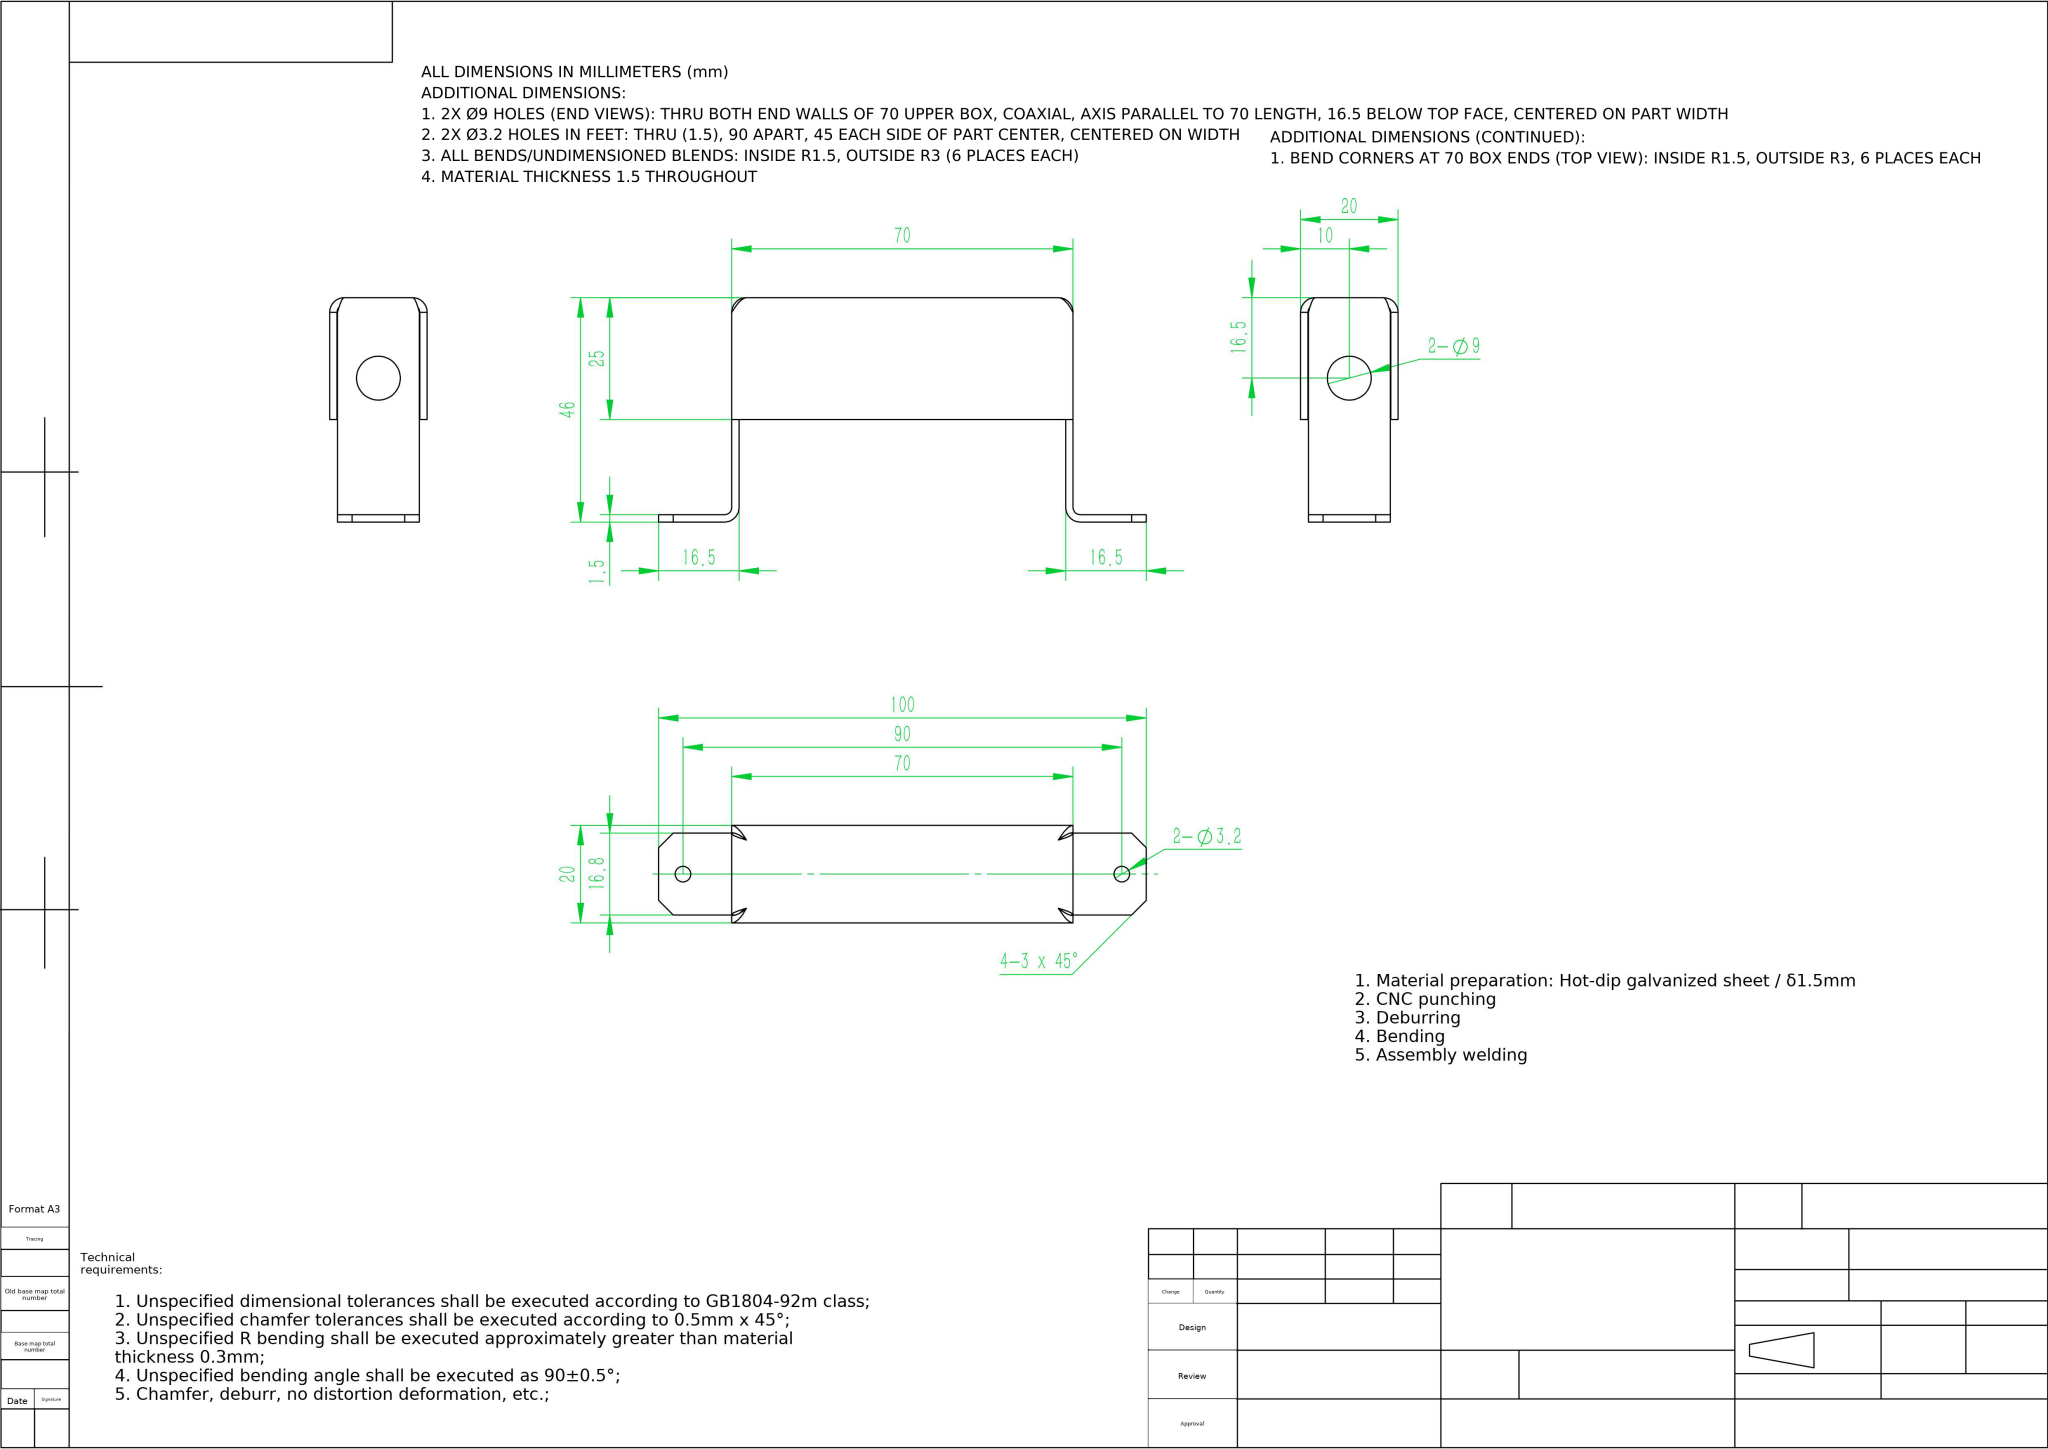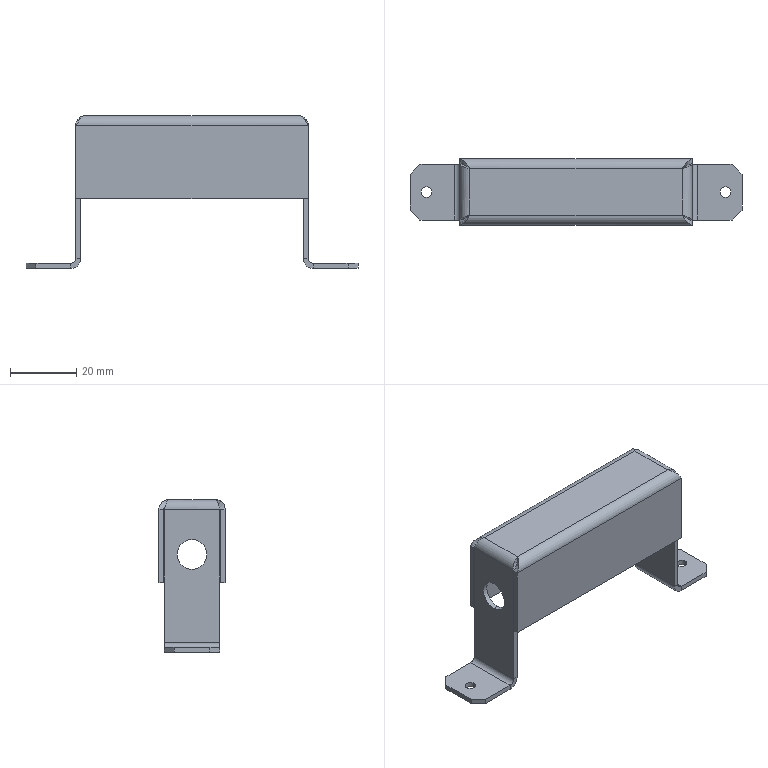Part | NX | mm | 1 solid | 66 faces | box 100 x 20 x 46 mm | volume 9471 mm3 | plane 38 | cylinder 20 | spline 8 | commonest cylinder face diameters 3 x6 6 x6 9 x4 3.2 x4